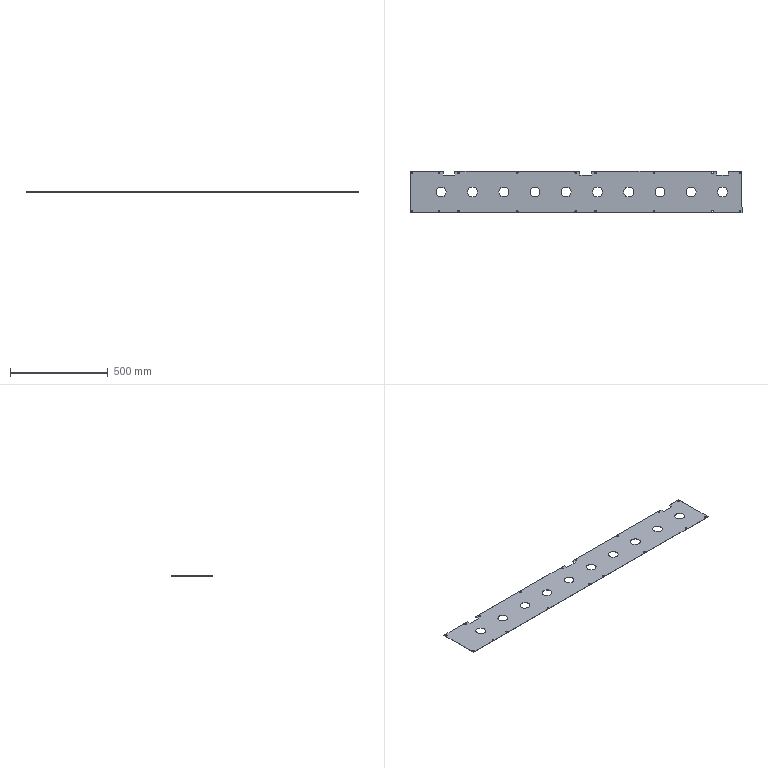Component | SolidWorks | CableCompartmentPartition-1 | 1 solid | 74 faces | box 1700 x 213 x 1.2 mm | volume 405412 mm3 | cylinder 56 | plane 18 | commonest cylinder face diameters 8.5 x36 50 x20
build123d program:
from build123d import *

# Parameters (mm, degrees)
SKETCH1_R      = 4.25
SKETCH1_R_2    = 25
EXTRUDE1_DEPTH = 1.2


with BuildPart() as part:
    # Sketch1 → Extrude1 (new body)
    with BuildSketch(Plane.XY):
        Polygon((-121.714, -2967.841), (-121.714, -2987.841), (-181.714, -2987.841), (-181.714, -2967.841), (-821.714, -2967.841), (-821.714, -2987.841), (-881.714, -2987.841), (-881.714, -2967.841), (-1521.714, -2967.841), (-1521.714, -2987.841), (-1581.714, -2987.841), (-1581.714, -2967.841), (-1651.714, -2967.841), (-1651.714, -3180.841), (48.286, -3180.841), (48.286, -2967.841), align=None)
        with Locations((-1640.714, -3173.341)):
            Circle(SKETCH1_R, mode=Mode.SUBTRACT)
        with Locations((-1500.714, -3173.341)):
            Circle(SKETCH1_R, mode=Mode.SUBTRACT)
        with Locations((-1200.714, -3173.341)):
            Circle(SKETCH1_R, mode=Mode.SUBTRACT)
        with Locations((-900.714, -3173.341)):
            Circle(SKETCH1_R, mode=Mode.SUBTRACT)
        with Locations((-800.714, -3173.341)):
            Circle(SKETCH1_R, mode=Mode.SUBTRACT)
        with Locations((-500.714, -3173.341)):
            Circle(SKETCH1_R, mode=Mode.SUBTRACT)
        with Locations((-200.714, -3173.341)):
            Circle(SKETCH1_R, mode=Mode.SUBTRACT)
        with Locations((-100.714, -3173.341)):
            Circle(SKETCH1_R, mode=Mode.SUBTRACT)
        with Locations((39.286, -3173.341)):
            Circle(SKETCH1_R, mode=Mode.SUBTRACT)
        with Locations((-1551.714, -3074.341)):
            Circle(SKETCH1_R_2, mode=Mode.SUBTRACT)
        with Locations((-1391.714, -3074.341)):
            Circle(SKETCH1_R_2, mode=Mode.SUBTRACT)
        with Locations((-1231.714, -3074.341)):
            Circle(SKETCH1_R_2, mode=Mode.SUBTRACT)
        with Locations((-1071.714, -3074.341)):
            Circle(SKETCH1_R_2, mode=Mode.SUBTRACT)
        with Locations((-911.714, -3074.341)):
            Circle(SKETCH1_R_2, mode=Mode.SUBTRACT)
        with Locations((-1640.714, -2975.341)):
            Circle(SKETCH1_R, mode=Mode.SUBTRACT)
        with Locations((-1500.714, -2975.341)):
            Circle(SKETCH1_R, mode=Mode.SUBTRACT)
        with Locations((-1200.714, -2975.341)):
            Circle(SKETCH1_R, mode=Mode.SUBTRACT)
        with Locations((-900.714, -2975.341)):
            Circle(SKETCH1_R, mode=Mode.SUBTRACT)
        with Locations((-751.714, -3074.341)):
            Circle(SKETCH1_R_2, mode=Mode.SUBTRACT)
        with Locations((-591.714, -3074.341)):
            Circle(SKETCH1_R_2, mode=Mode.SUBTRACT)
        with Locations((-431.714, -3074.341)):
            Circle(SKETCH1_R_2, mode=Mode.SUBTRACT)
        with Locations((-271.714, -3074.341)):
            Circle(SKETCH1_R_2, mode=Mode.SUBTRACT)
        with Locations((-111.714, -3074.341)):
            Circle(SKETCH1_R_2, mode=Mode.SUBTRACT)
        with Locations((-800.714, -2975.341)):
            Circle(SKETCH1_R, mode=Mode.SUBTRACT)
        with Locations((-500.714, -2975.341)):
            Circle(SKETCH1_R, mode=Mode.SUBTRACT)
        with Locations((-200.714, -2975.341)):
            Circle(SKETCH1_R, mode=Mode.SUBTRACT)
        with Locations((-100.714, -2975.341)):
            Circle(SKETCH1_R, mode=Mode.SUBTRACT)
        with Locations((39.286, -2975.341)):
            Circle(SKETCH1_R, mode=Mode.SUBTRACT)
    extrude(amount=EXTRUDE1_DEPTH)


solid = part.part

# Placed as in the assembly
solid = solid.moved(Location((-1848.644, 2980.948, -80), (-180, 0, 180)))